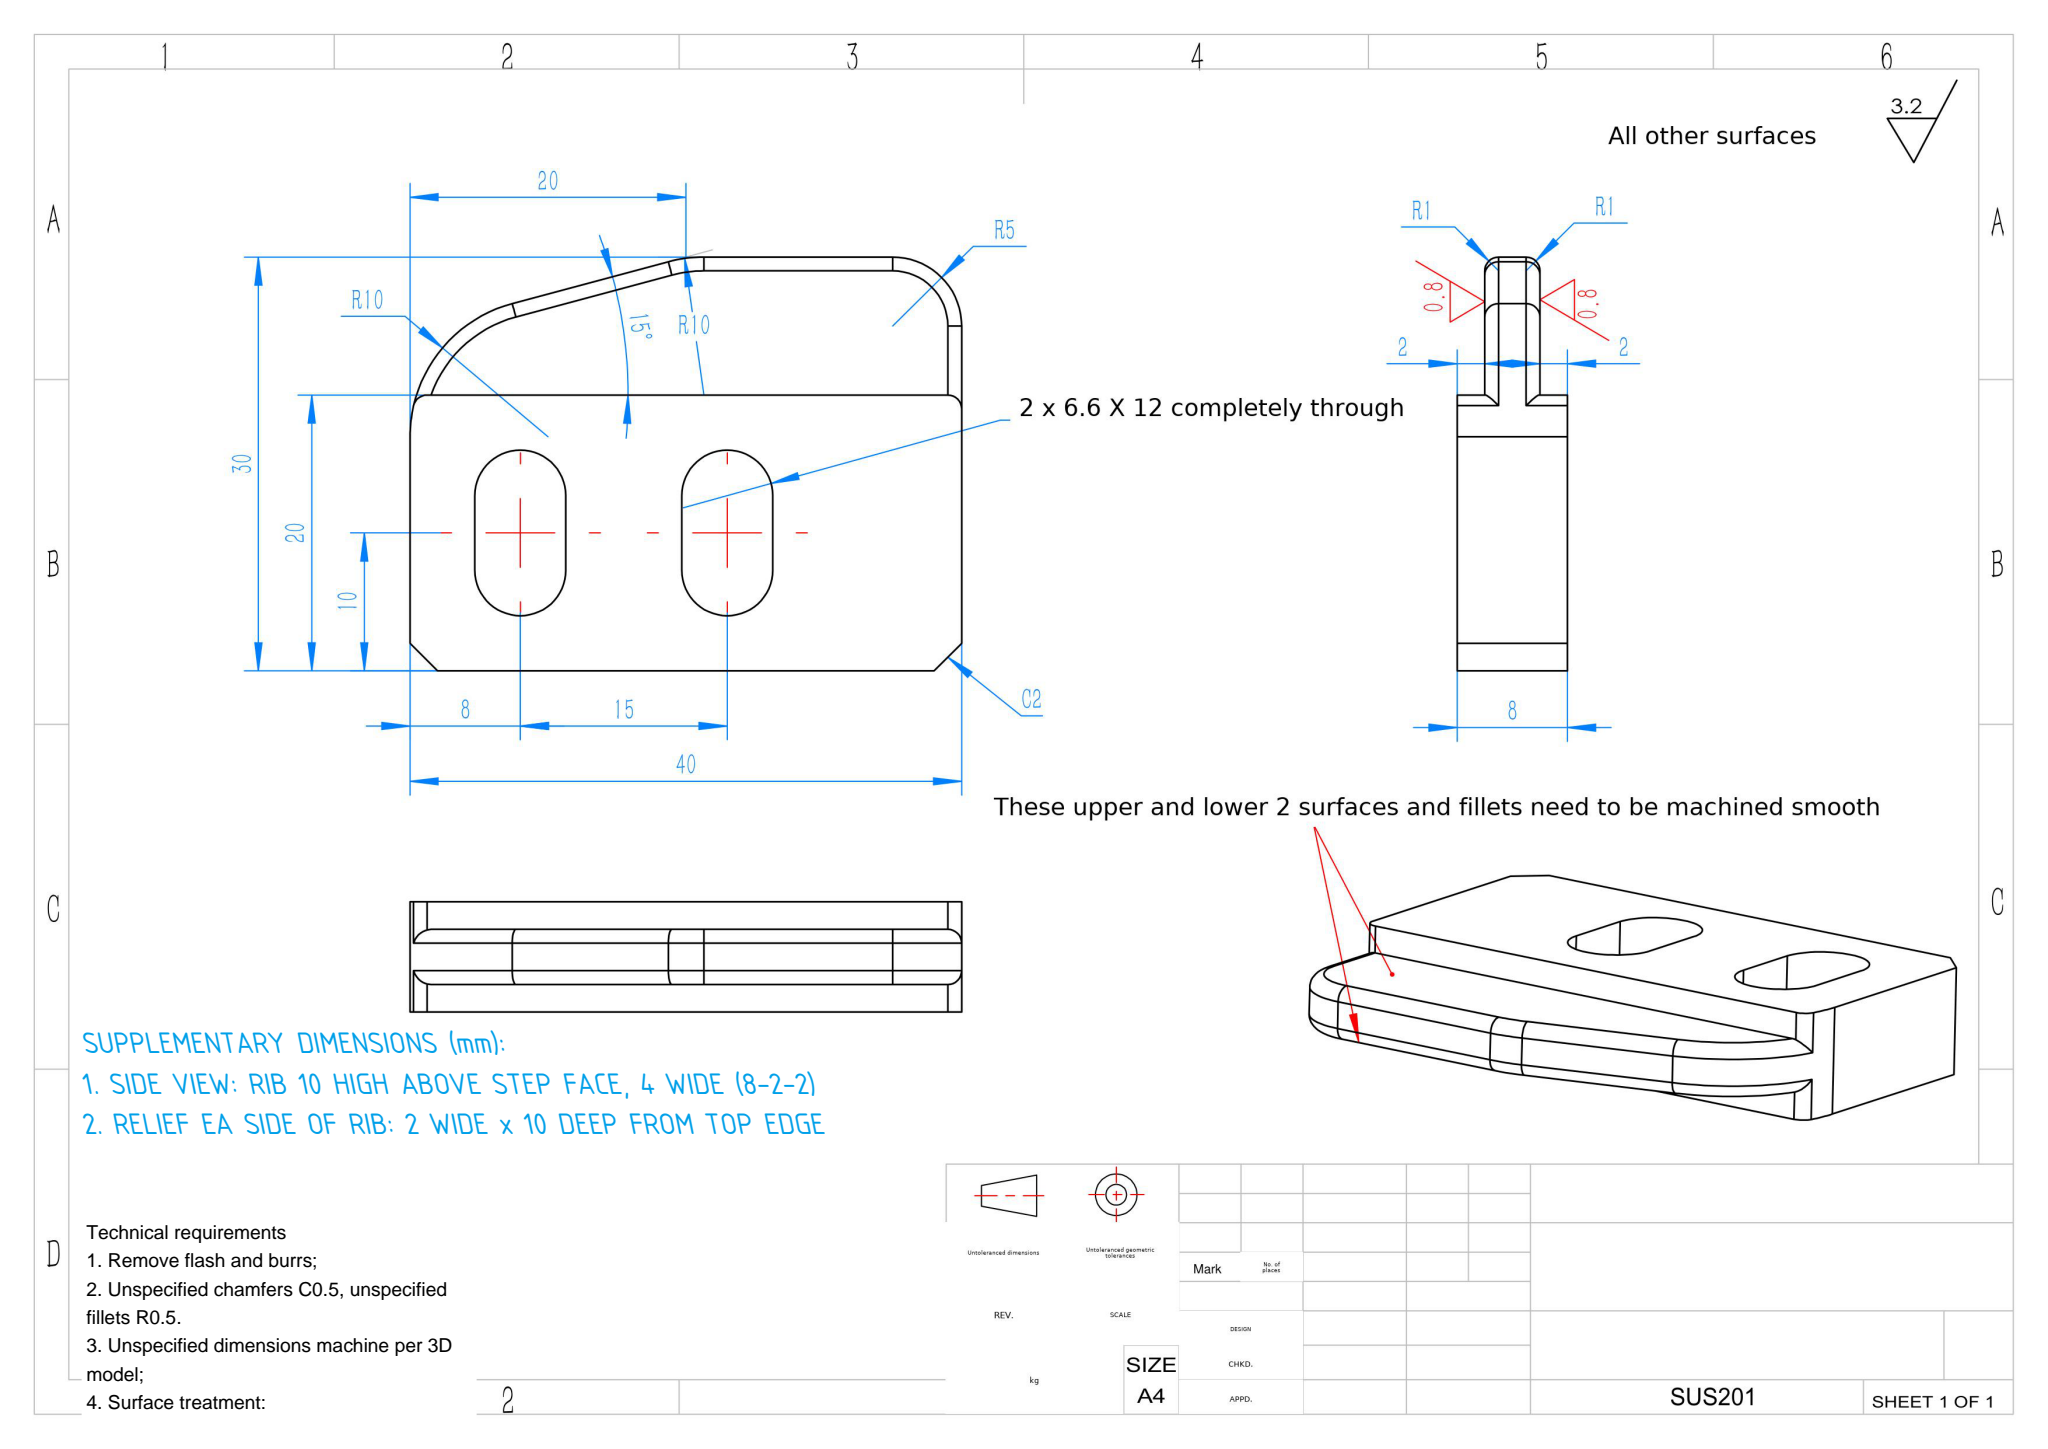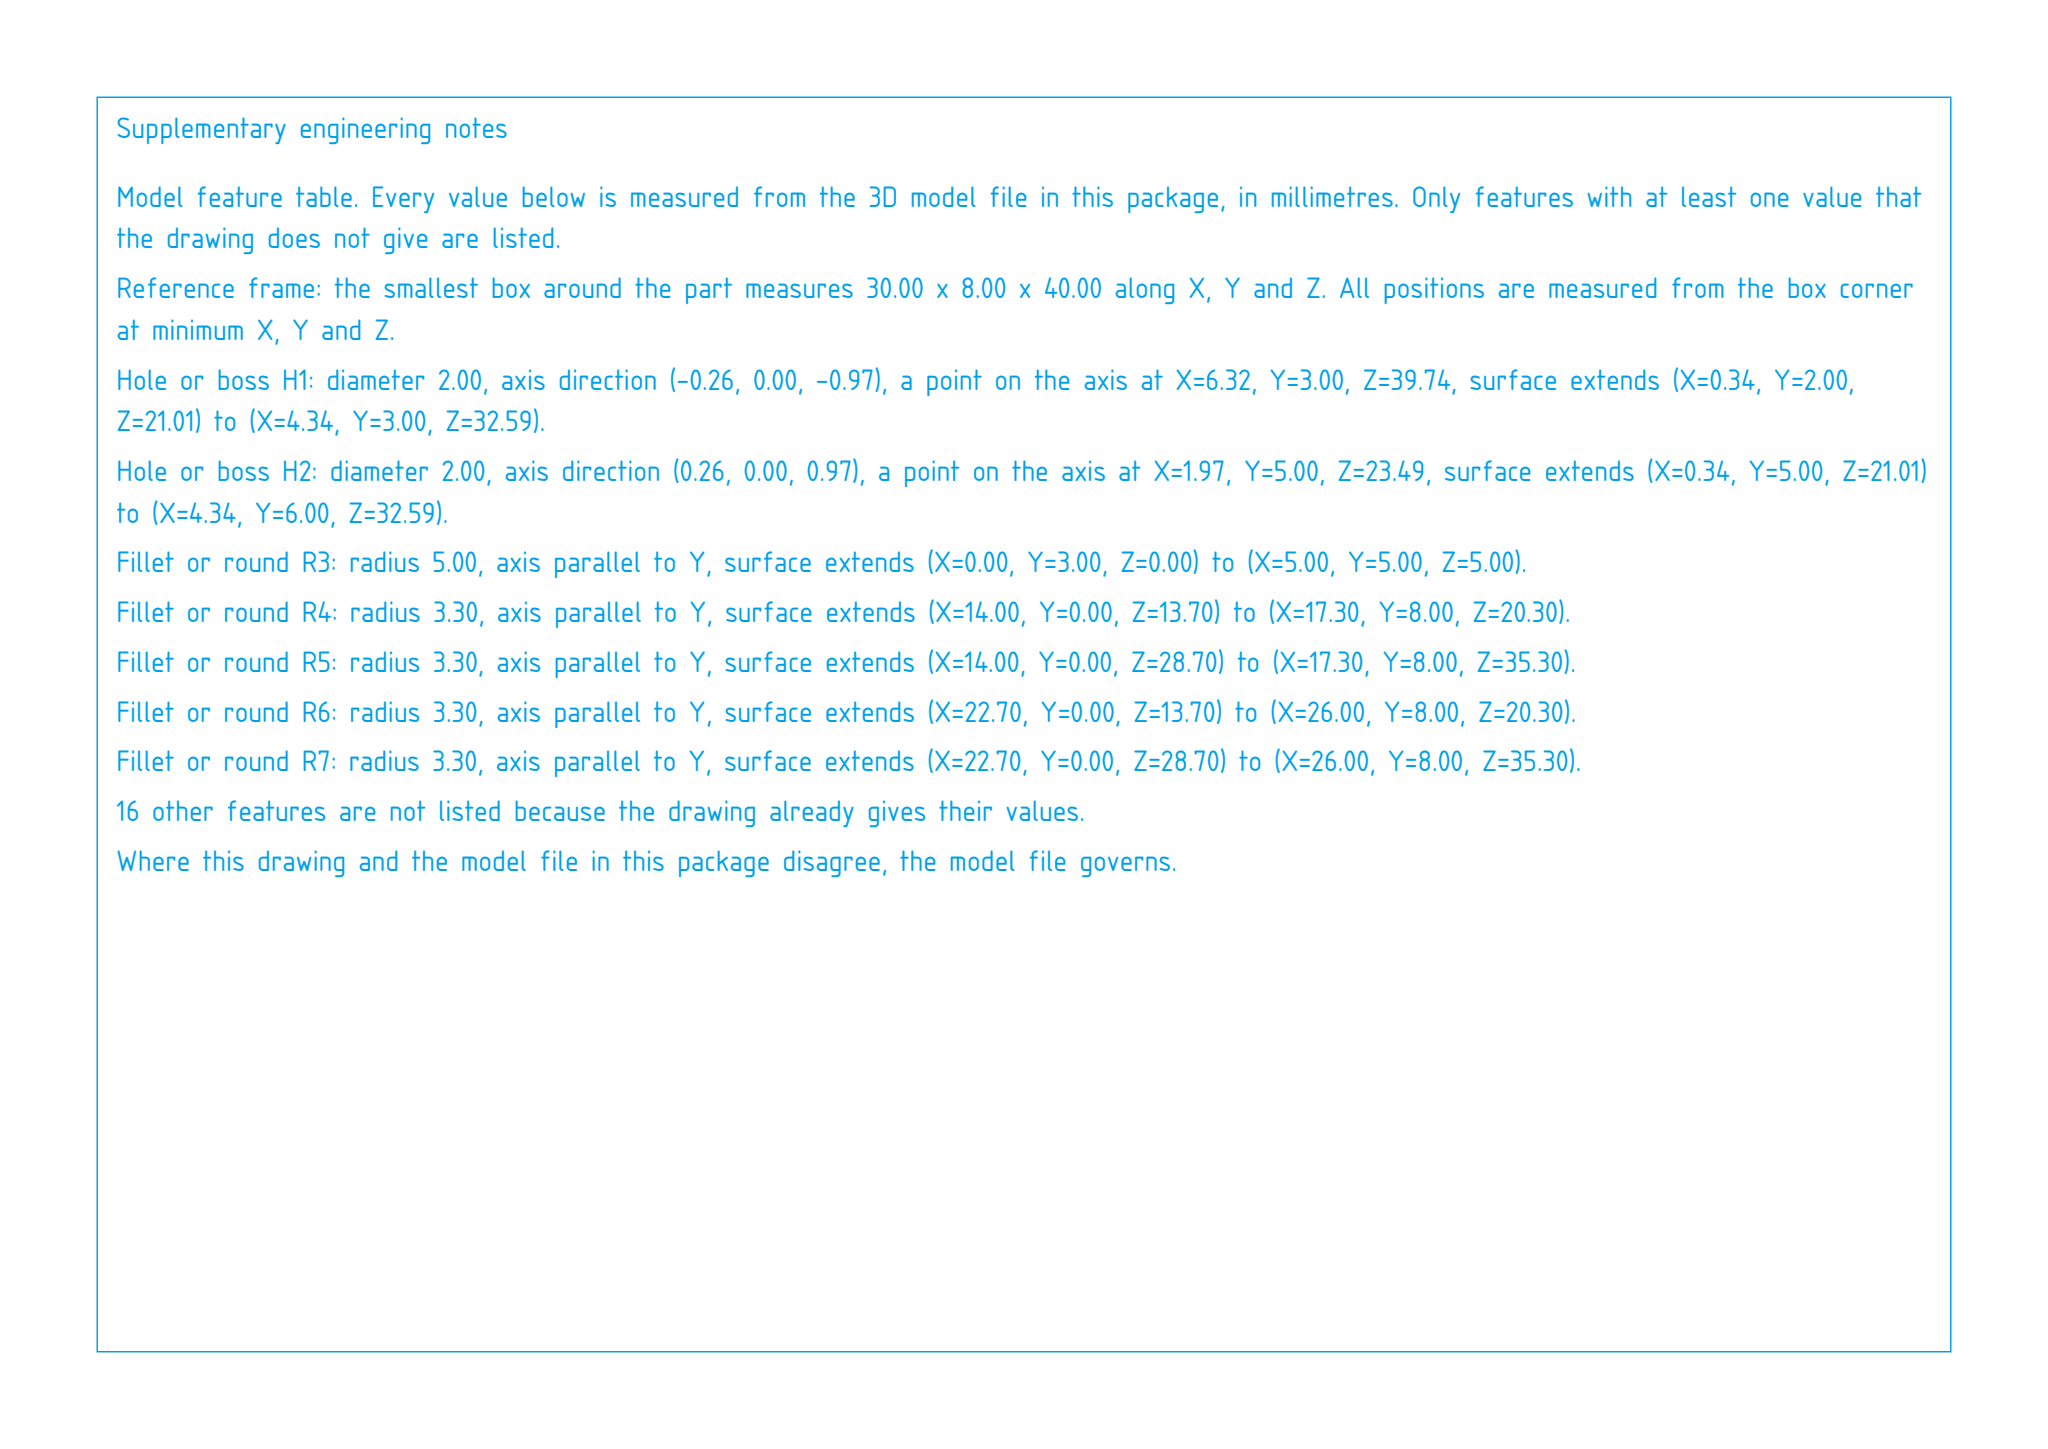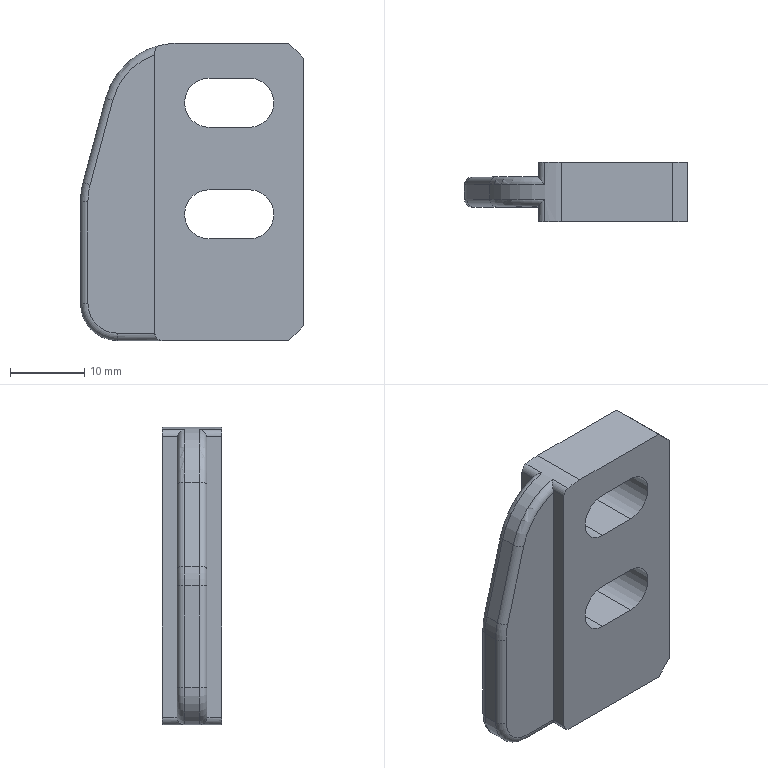Part | SolidWorks | mm | 1 solid | 40 faces | box 30 x 8 x 40 mm | volume 6544 mm3 | plane 17 | cylinder 17 | torus 6 | commonest cylinder face diameters 2 x10 6.6 x4 20 x2 10 x1